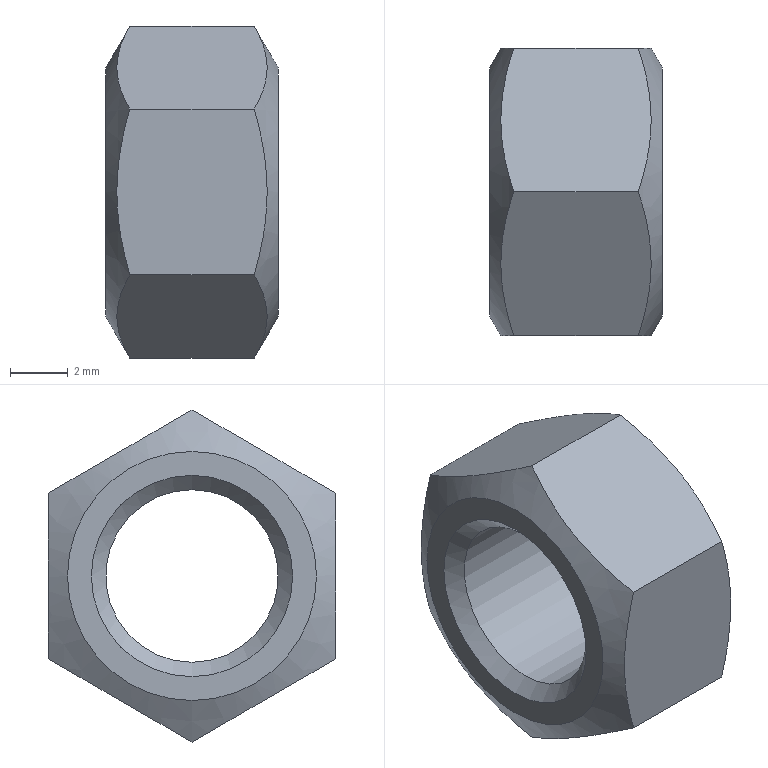Component | NX | NUT_2 | 1 solid | 13 faces | volume 329 mm3 | plane 8 | cone 4 | cylinder 1 | commonest cylinder face diameters 6 x1